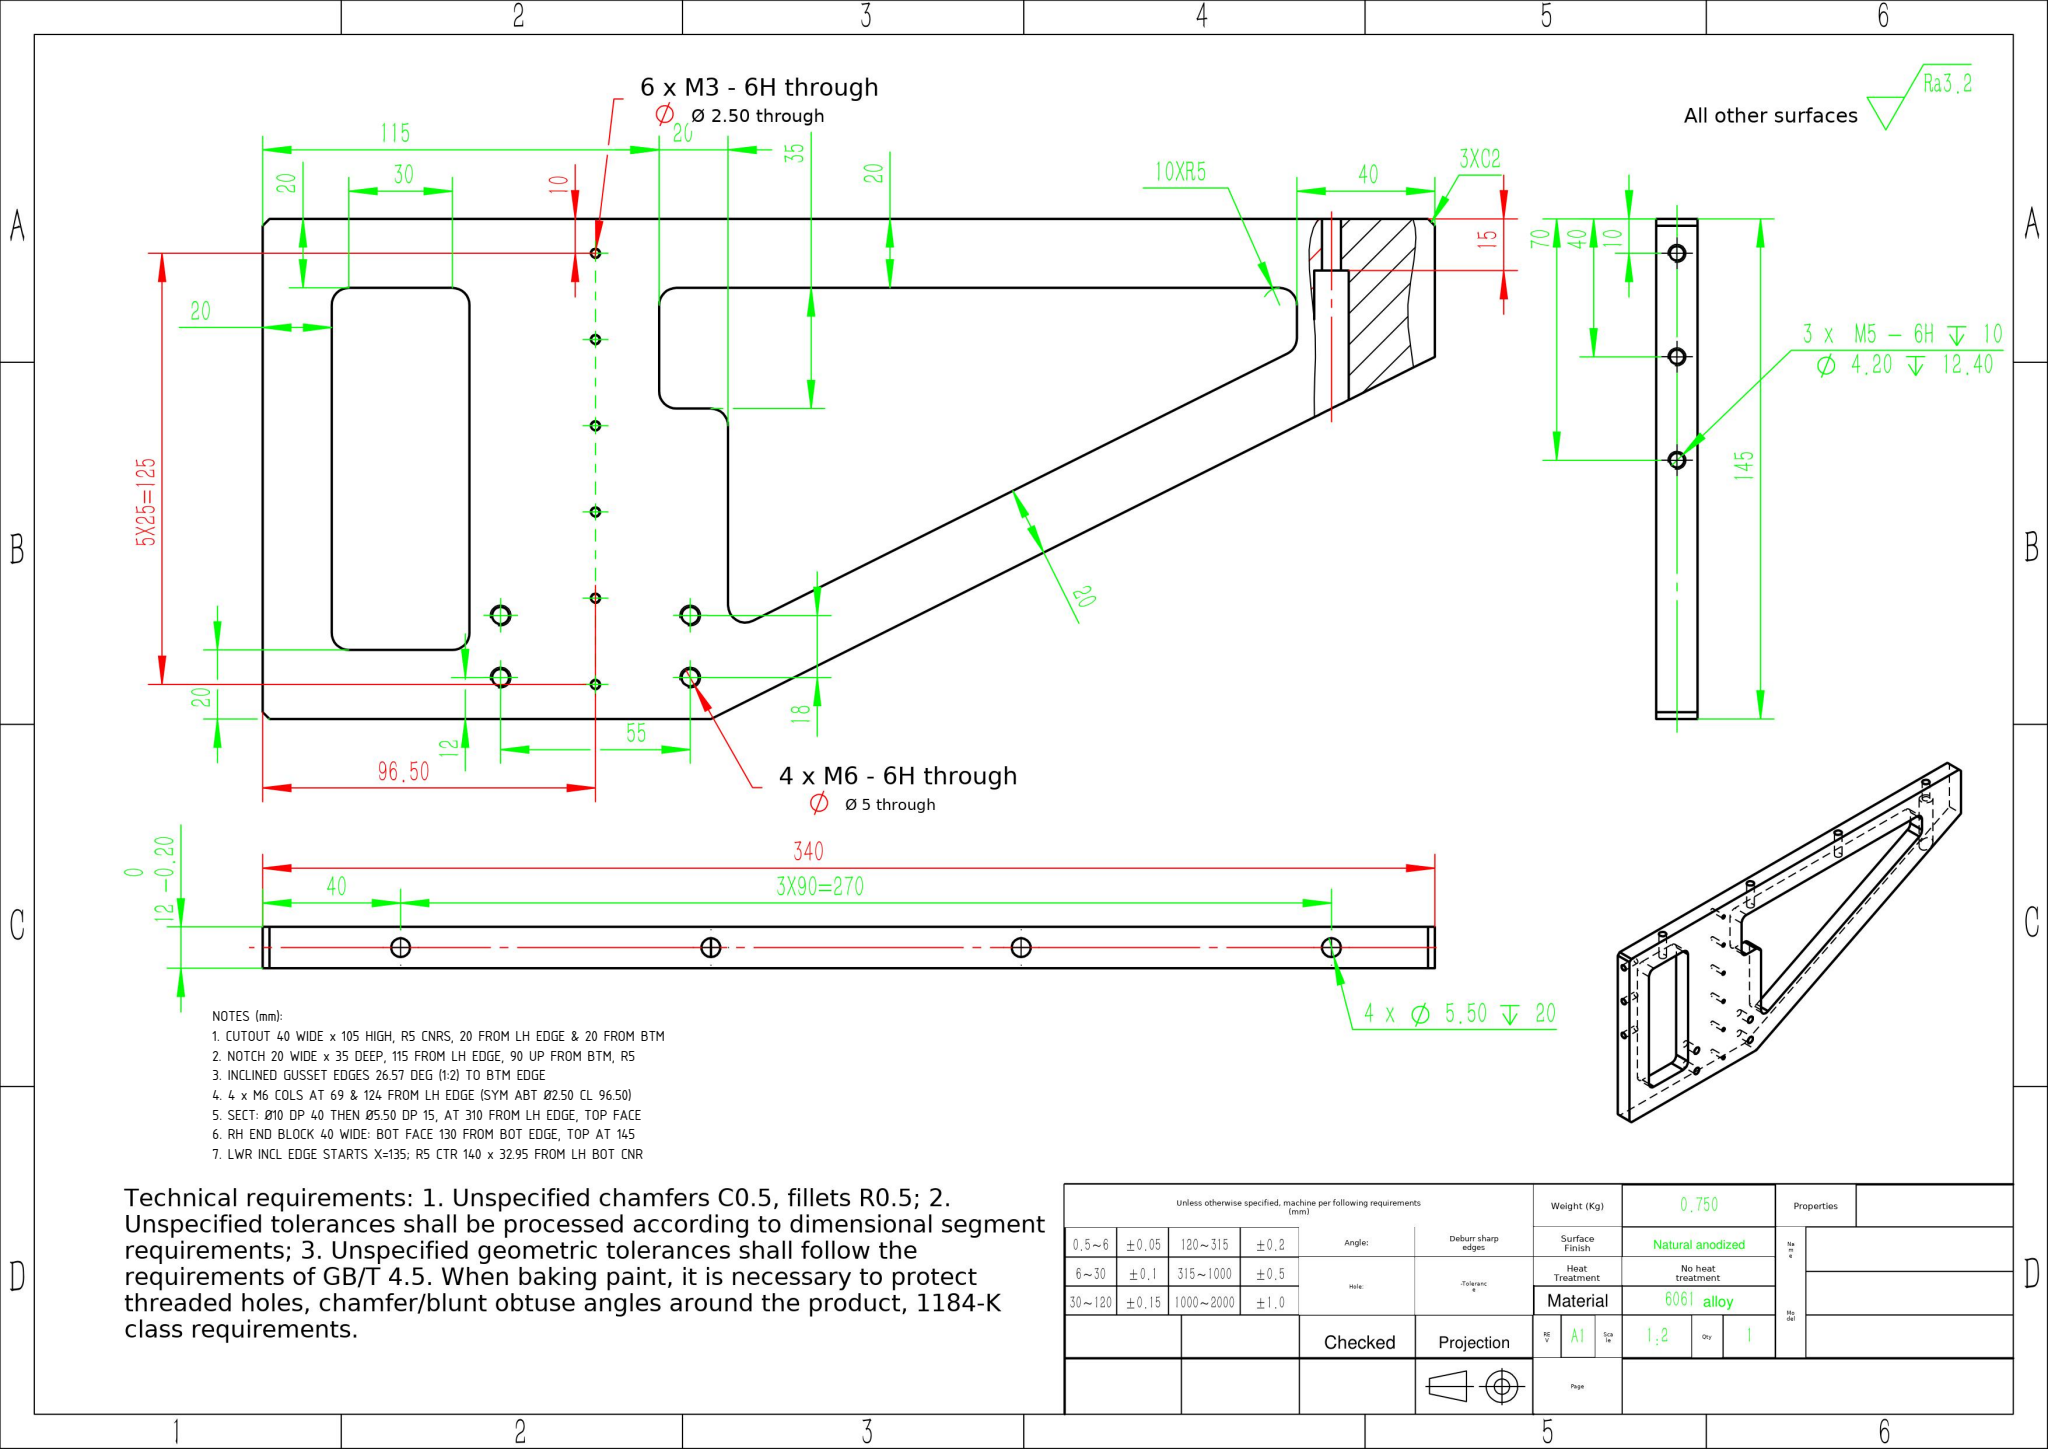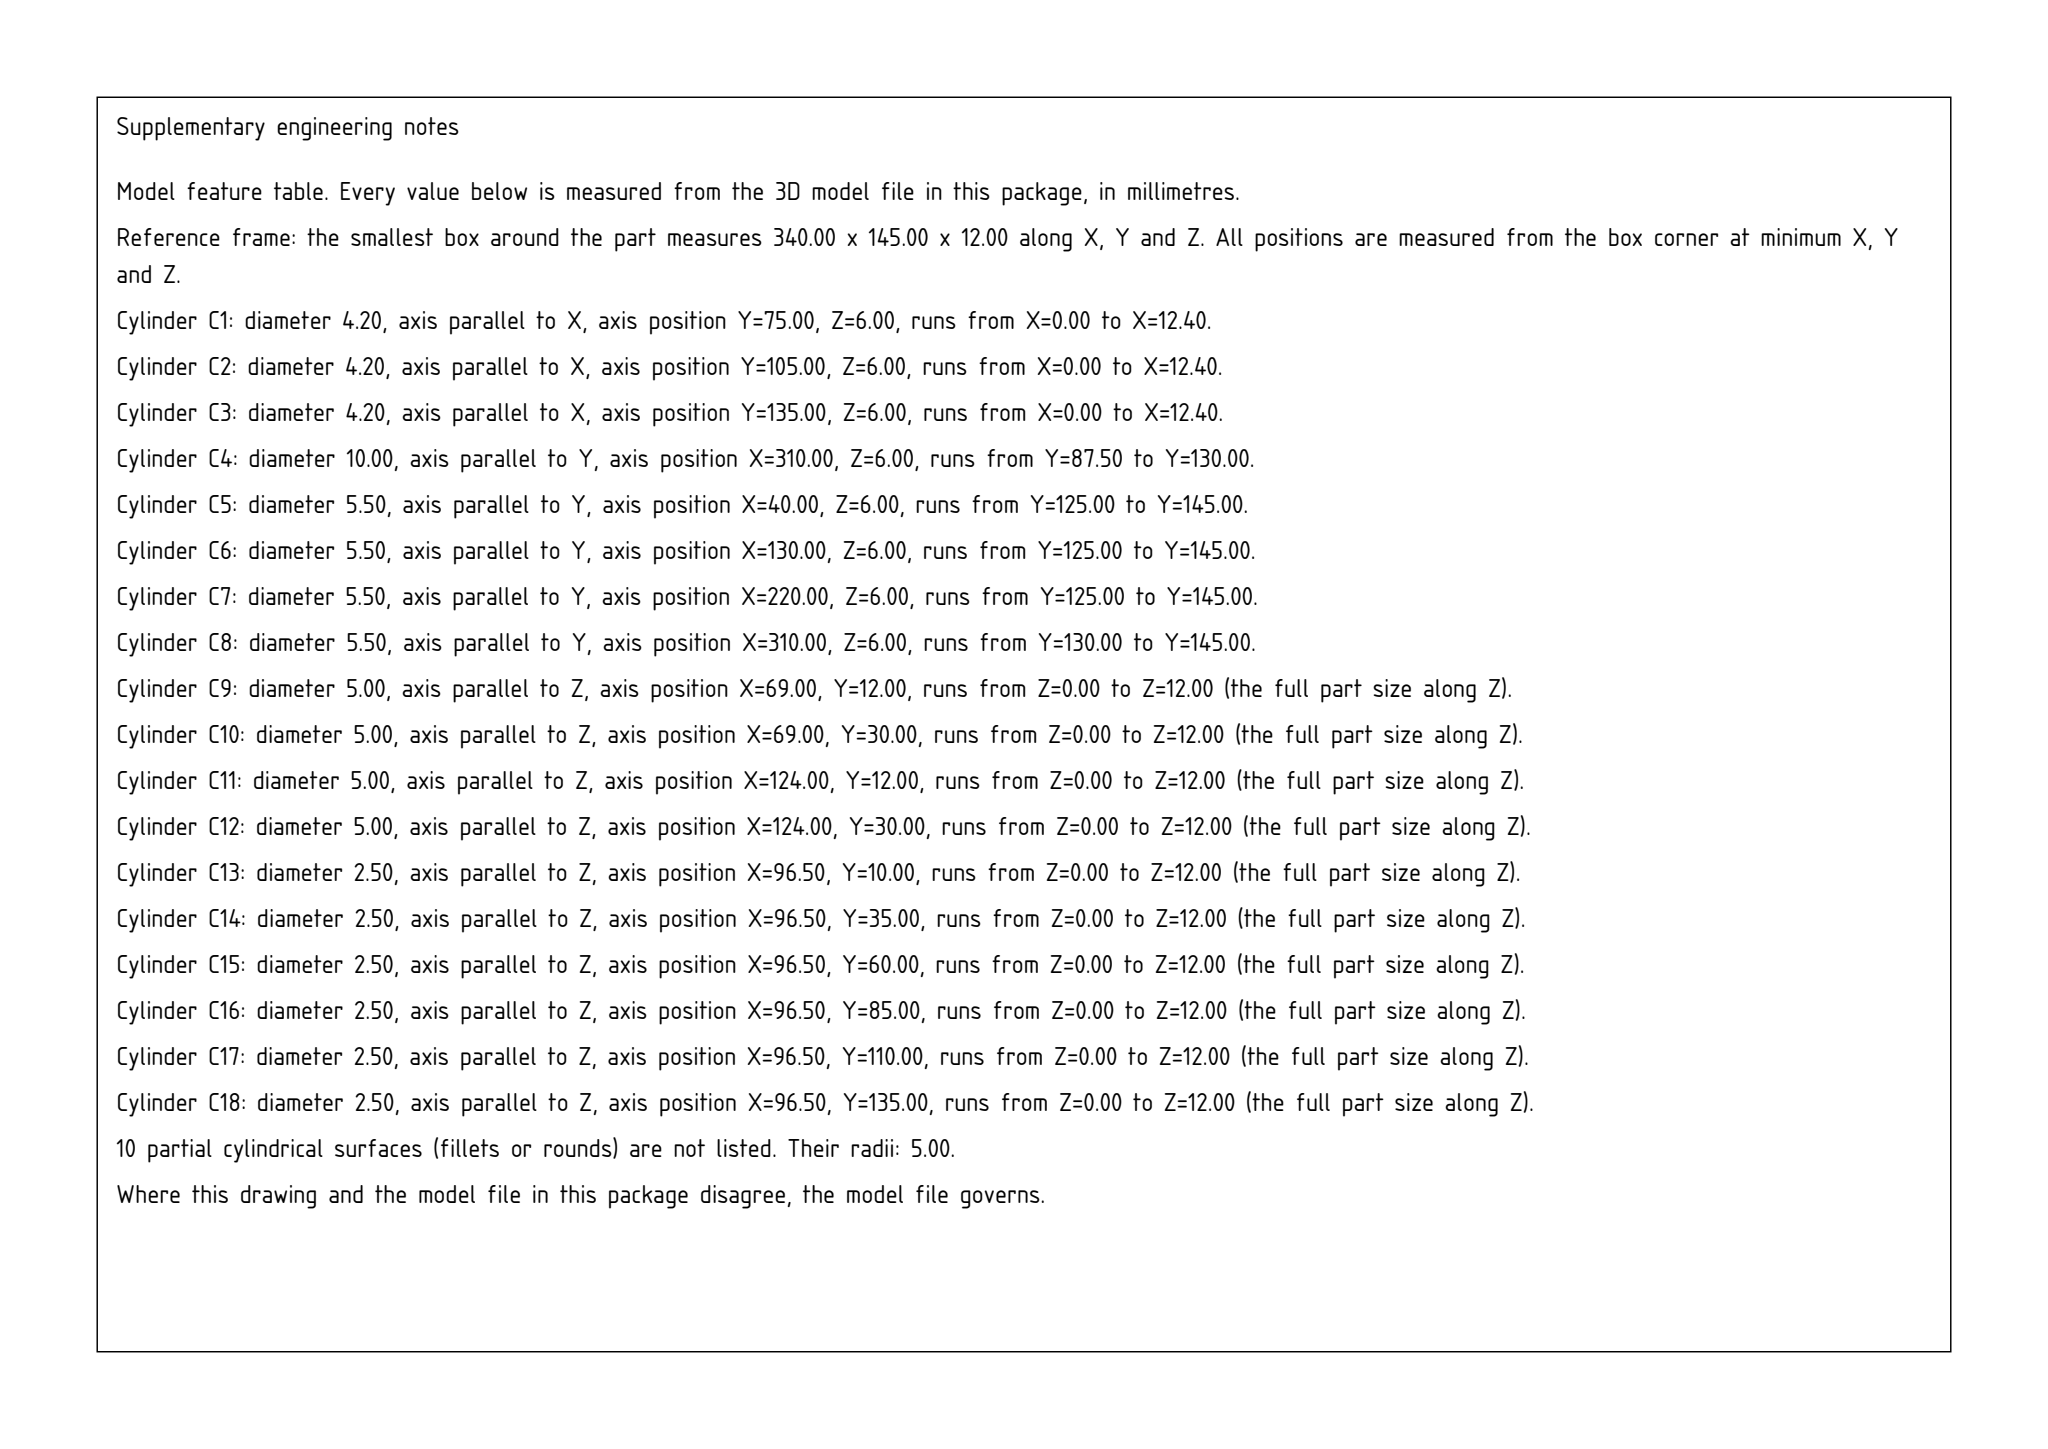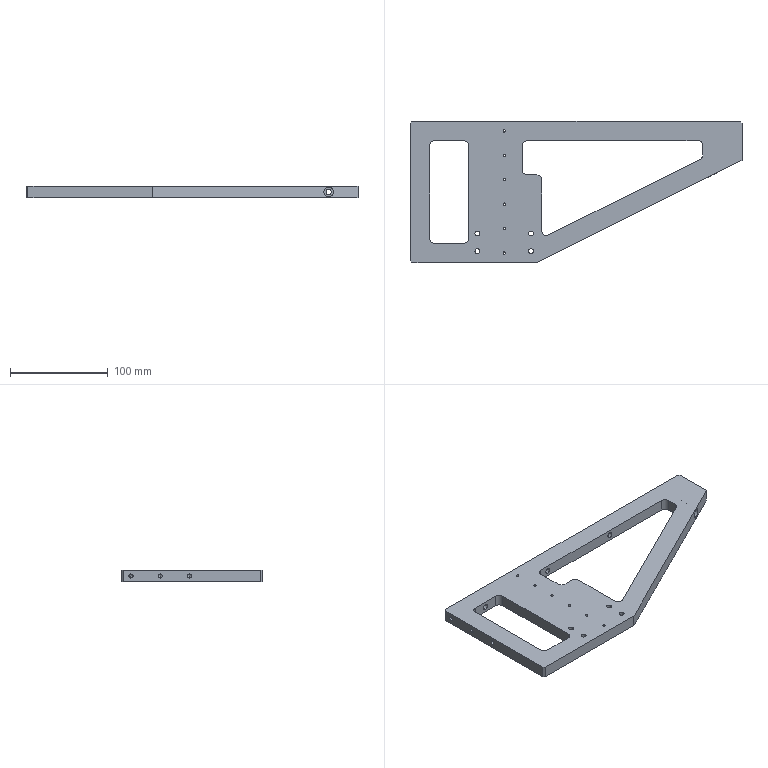Part | SolidWorks | mm | 1 solid | 73 faces | box 340 x 145 x 12 mm | volume 277661 mm3 | cylinder 46 | plane 21 | cone 6 | commonest cylinder face diameters 2.5 x12 10 x12 5 x8 5.5 x8 4.2 x6
Drawing notes:
CUTOUT 40 WIDE x 105 HIGH, R5 CNRS, 20 FROM LH EDGE & 20 FROM BTM | from the solid: R5 cyls dia10 z at (25,25),(55,25),(25,120),(55,120); planes x=20/60, y=20/125
NOTCH 20 WIDE x 35 DEEP, 115 FROM LH EDGE, 90 UP FROM BTM, R5 | from the solid: planes x=115,x=135,y=90,y=125; R5 cyls at (120,120),(120,95),(130,85)
INCLINED GUSSET EDGES 26.57 DEG (1:2) TO BTM EDGE | from the solid: R5 tangent cyls (140,32.95) & (295,110.45): dy/dx=77.5/155=0.500 -> 26.57 deg
4 x M6 COLS AT 69 & 124 FROM LH EDGE (SYM ABT Ø2.50 CL 96.50) | from the solid: Ø5.0 z-holes at x=69.0 and x=124.0 (y=12 & 30); Ø2.5 col at x=96.5
SECT: Ø10 DP 40 THEN Ø5.50 DP 15, AT 310 FROM LH EDGE, TOP FACE | from the solid: Ø10 y-axis cyl at [310,-,6] len 40; Ø5.5 y-axis at [310,-,6] len 15
RH END BLOCK 40 WIDE: BOT FACE 130 FROM BOT EDGE, TOP AT 145 | from the solid: x-planes 300 & 340 (40 wide); y-planes 130 and 145; 145-130=15
LWR INCL EDGE STARTS X=135; R5 CTR 140 x 32.95 FROM LH BOT CNR | from the solid: x-plane 135; R5 (Ø10 z) fillet cyl at [140, 32.95]
build123d program:
from build123d import *

# Parameters (mm, degrees)
BOSS_EXTRUDE1_DEPTH                               = 6
CUT_EXTRUDE1_DEPTH                                = 370.823
M5_CLEARANCE_HOLE1_D                              = 5.5
M5_CLEARANCE_HOLE1_DEPTH                          = 20
M5_CLEARANCE_HOLE1_TIP                            = 1.652
M5_TAPPED_HOLE1_D                                 = 4.2
M5_TAPPED_HOLE1_DEPTH                             = 12.4
M5_TAPPED_HOLE1_TIP                               = 1.262
HOLE_SIZE_ACCORDING_TO_TYPE_1_OF_HEXA_D           = 5.5
HOLE_SIZE_ACCORDING_TO_TYPE_1_OF_HEXA_CBORE_D     = 10
HOLE_SIZE_ACCORDING_TO_TYPE_1_OF_HEXA_CBORE_DEPTH = 130
M3_TAPPED_HOLE1_D                                 = 2.5
M6_TAPPED_HOLE1_D                                 = 5
CHAMFER1_SIZE                                     = 2


with BuildPart() as part:
    # Sketch1 → Boss-Extrude1 (new, symmetric)
    with BuildSketch(Plane.XY):
        Polygon((0, 0), (0, 145), (340, 145), (340, 105), (130, 0), align=None)
    extrude(amount=BOSS_EXTRUDE1_DEPTH, both=True)

    # Sketch9 → Cut-Extrude1 (cut, through all)
    with BuildSketch(Plane.XY.offset(6)):
        with BuildLine():
            Line((142.236, 28.479), (297.236, 105.979))
            ThreePointArc((297.236, 105.979), (299.253, 107.822), (300, 110.451))
            Line((300, 110.451), (300, 120))
            ThreePointArc((300, 120), (298.536, 123.536), (295, 125))
            Line((295, 125), (120, 125))
            ThreePointArc((120, 125), (116.464, 123.536), (115, 120))
            Line((115, 120), (115, 95))
            ThreePointArc((115, 95), (116.464, 91.464), (120, 90))
            Line((120, 90), (130, 90))
            ThreePointArc((130, 90), (133.536, 88.536), (135, 85))
            Line((135, 85), (135, 32.951))
            ThreePointArc((135, 32.951), (137.371, 28.698), (142.236, 28.479))
        make_face()
        with BuildLine():
            Line((20, 120), (20, 25))
            ThreePointArc((20, 25), (21.464, 21.464), (25, 20))
            Line((25, 20), (55, 20))
            ThreePointArc((55, 20), (58.536, 21.464), (60, 25))
            Line((60, 25), (60, 120))
            ThreePointArc((60, 120), (58.536, 123.536), (55, 125))
            Line((55, 125), (25, 125))
            ThreePointArc((25, 125), (21.464, 123.536), (20, 120))
        make_face()
    extrude(amount=-CUT_EXTRUDE1_DEPTH, mode=Mode.SUBTRACT)

    # M5 Clearance Hole1
    with Locations(Plane(origin=(0, 145, 0), x_dir=(1, 0, 0), z_dir=(0, 1, 0))):
        with Locations((40, 0), (130, 0), (220, 0), (310, 0)):
            Hole(M5_CLEARANCE_HOLE1_D / 2, depth=M5_CLEARANCE_HOLE1_DEPTH)
            with Locations((0, 0, -(M5_CLEARANCE_HOLE1_DEPTH + M5_CLEARANCE_HOLE1_TIP / 2))):  # 118° drill point
                Cone(0, M5_CLEARANCE_HOLE1_D / 2, M5_CLEARANCE_HOLE1_TIP, mode=Mode.SUBTRACT)

    # M5 Tapped Hole1
    with Locations(Plane.ZY):
        with Locations((0, 75), (0, 105), (0, 135)):
            Hole(M5_TAPPED_HOLE1_D / 2, depth=M5_TAPPED_HOLE1_DEPTH)
            with Locations((0, 0, -(M5_TAPPED_HOLE1_DEPTH + M5_TAPPED_HOLE1_TIP / 2))):  # 118° drill point
                Cone(0, M5_TAPPED_HOLE1_D / 2, M5_TAPPED_HOLE1_TIP, mode=Mode.SUBTRACT)

    # Hole Size _ According to_ Type 1 of Hexa (through all)
    with Locations(Plane(origin=(0, 0, 0), x_dir=(-1, 0, 0), z_dir=(0, -1, 0))):
        with Locations((-310, 0)):
            CounterBoreHole(HOLE_SIZE_ACCORDING_TO_TYPE_1_OF_HEXA_D / 2, HOLE_SIZE_ACCORDING_TO_TYPE_1_OF_HEXA_CBORE_D / 2, HOLE_SIZE_ACCORDING_TO_TYPE_1_OF_HEXA_CBORE_DEPTH)

    # M3 Tapped Hole1 (through all)
    with Locations(Plane.XY.offset(6)):
        with Locations((96.5, 135), (96.5, 110), (96.5, 85), (96.5, 60), (96.5, 35), (96.5, 10)):
            Hole(M3_TAPPED_HOLE1_D / 2)

    # M6 Tapped Hole1 (through all)
    with Locations(Plane.XY.offset(6)):
        with Locations((69, 30), (69, 12), (124, 30), (124, 12)):
            Hole(M6_TAPPED_HOLE1_D / 2)

    # Chamfer1
    chamfer1_edges = [part.edges().sort_by_distance(p)[0] for p in [
        (0, 0, 0),
        (0, 145, 0),
        (340, 145, 0),
    ]]
    chamfer(chamfer1_edges, length=CHAMFER1_SIZE)


solid = part.part